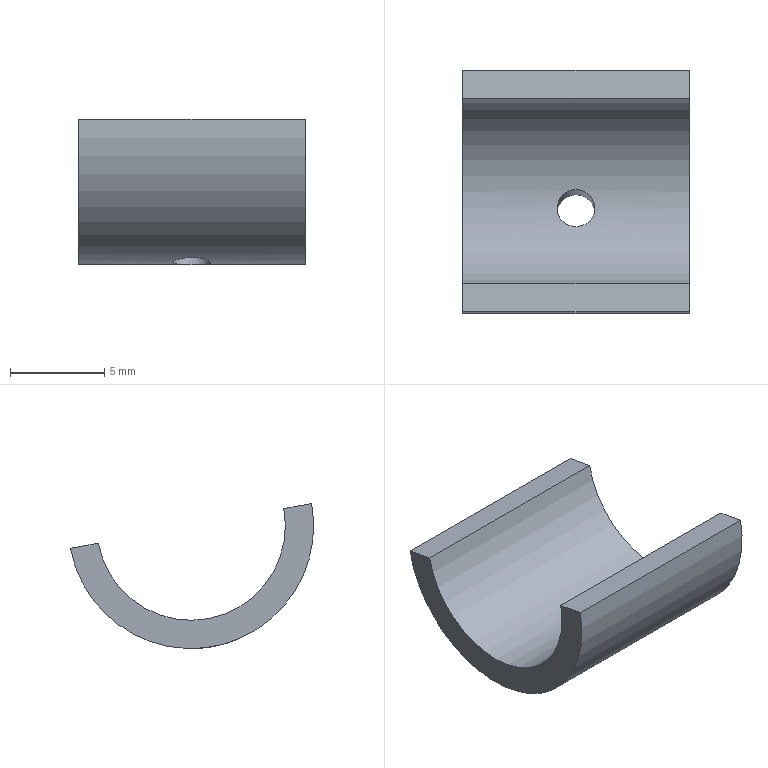Component | NX | 17C__27 | 1 solid | 7 faces | box 12 x 12.89 x 7.69 mm | volume 320 mm3 | plane 4 | cylinder 3 | commonest cylinder face diameters 10 x1 13 x1 2 x1
STEP:
#1=CARTESIAN_POINT('',(0.,0.,0.));
#2=DIRECTION('',(0.,0.,1.));
#3=DIRECTION('',(1.,0.,0.));
#4=AXIS2_PLACEMENT_3D('',#1,#2,#3);
#5=CARTESIAN_POINT('',(122.022,103.543,62.298));
#6=VERTEX_POINT('',#5);
#7=CARTESIAN_POINT('',(110.022,103.543,62.298));
#8=VERTEX_POINT('',#7);
#9=CARTESIAN_POINT('',(122.022,103.543,62.298));
#10=DIRECTION('',(-1.,0.,0.));
#11=VECTOR('',#10,1.);
#12=LINE('',#9,#11);
#13=CARTESIAN_POINT('',(122.022,98.628,63.213));
#14=DIRECTION('',(-1.,0.,0.));
#15=DIRECTION('',(0.,-0.183,-0.9831));
#16=AXIS2_PLACEMENT_3D('',#13,#14,#15);
#17=CYLINDRICAL_SURFACE('',#16,5.);
#18=CARTESIAN_POINT('',(-1.571,0.));
#19=DIRECTION('',(0.,1.));
#20=VECTOR('',#19,1.);
#21=LINE('',#18,#20);
#22=(GEOMETRIC_REPRESENTATION_CONTEXT(2)PARAMETRIC_REPRESENTATION_CONTEXT()REPRESENTATION_CONTEXT('',''));
#23=DEFINITIONAL_REPRESENTATION('',(#21),#22);
#24=PCURVE('',#17,#23);
#25=CARTESIAN_POINT('',(122.022,105.018,62.023));
#26=DIRECTION('',(0.,-0.183,-0.9831));
#27=DIRECTION('',(0.,-0.9831,0.183));
#28=AXIS2_PLACEMENT_3D('',#25,#26,#27);
#29=PLANE('',#28);
#30=CARTESIAN_POINT('',(1.5,0.));
#31=DIRECTION('',(0.,1.));
#32=VECTOR('',#31,1.);
#33=LINE('',#30,#32);
#34=(GEOMETRIC_REPRESENTATION_CONTEXT(2)PARAMETRIC_REPRESENTATION_CONTEXT()REPRESENTATION_CONTEXT('',''));
#35=DEFINITIONAL_REPRESENTATION('',(#33),#34);
#36=PCURVE('',#29,#35);
#37=SURFACE_CURVE('',#12,(#24,#36),.PCURVE_S1.);
#38=EDGE_CURVE('',#6,#8,#37,.T.);
#39=ORIENTED_EDGE('',*,*,#38,.F.);
#40=CARTESIAN_POINT('',(122.022,93.712,64.128));
#41=VERTEX_POINT('',#40);
#42=CARTESIAN_POINT('',(122.022,98.628,63.213));
#43=DIRECTION('',(-1.,0.,0.));
#44=DIRECTION('',(0.,-0.9831,0.183));
#45=AXIS2_PLACEMENT_3D('',#42,#43,#44);
#46=CIRCLE('',#45,5.);
#47=CARTESIAN_POINT('',(-4.712,0.));
#48=DIRECTION('',(1.,0.));
#49=VECTOR('',#48,1.);
#50=LINE('',#47,#49);
#51=(GEOMETRIC_REPRESENTATION_CONTEXT(2)PARAMETRIC_REPRESENTATION_CONTEXT()REPRESENTATION_CONTEXT('',''));
#52=DEFINITIONAL_REPRESENTATION('',(#50),#51);
#53=PCURVE('',#17,#52);
#54=CARTESIAN_POINT('',(122.022,98.628,63.213));
#55=DIRECTION('',(-1.,0.,0.));
#56=DIRECTION('',(0.,-0.183,-0.9831));
#57=AXIS2_PLACEMENT_3D('',#54,#55,#56);
#58=PLANE('',#57);
#59=CARTESIAN_POINT('',(0.,0.));
#60=DIRECTION('',(0.,1.));
#61=AXIS2_PLACEMENT_2D('',#59,#60);
#62=CIRCLE('',#61,5.);
#63=(GEOMETRIC_REPRESENTATION_CONTEXT(2)PARAMETRIC_REPRESENTATION_CONTEXT()REPRESENTATION_CONTEXT('',''));
#64=DEFINITIONAL_REPRESENTATION('',(#62),#63);
#65=PCURVE('',#58,#64);
#66=SURFACE_CURVE('',#46,(#53,#65),.PCURVE_S1.);
#67=EDGE_CURVE('',#6,#41,#66,.T.);
#68=ORIENTED_EDGE('',*,*,#67,.T.);
#69=CARTESIAN_POINT('',(110.022,93.712,64.128));
#70=VERTEX_POINT('',#69);
#71=CARTESIAN_POINT('',(122.022,93.712,64.128));
#72=DIRECTION('',(-1.,0.,0.));
#73=VECTOR('',#72,1.);
#74=LINE('',#71,#73);
#75=CARTESIAN_POINT('',(1.571,0.));
#76=DIRECTION('',(0.,1.));
#77=VECTOR('',#76,1.);
#78=LINE('',#75,#77);
#79=(GEOMETRIC_REPRESENTATION_CONTEXT(2)PARAMETRIC_REPRESENTATION_CONTEXT()REPRESENTATION_CONTEXT('',''));
#80=DEFINITIONAL_REPRESENTATION('',(#78),#79);
#81=PCURVE('',#17,#80);
#82=CARTESIAN_POINT('',(122.022,93.712,64.128));
#83=DIRECTION('',(0.,-0.183,-0.9831));
#84=DIRECTION('',(0.,-0.9831,0.183));
#85=AXIS2_PLACEMENT_3D('',#82,#83,#84);
#86=PLANE('',#85);
#87=CARTESIAN_POINT('',(0.,0.));
#88=DIRECTION('',(0.,1.));
#89=VECTOR('',#88,1.);
#90=LINE('',#87,#89);
#91=(GEOMETRIC_REPRESENTATION_CONTEXT(2)PARAMETRIC_REPRESENTATION_CONTEXT()REPRESENTATION_CONTEXT('',''));
#92=DEFINITIONAL_REPRESENTATION('',(#90),#91);
#93=PCURVE('',#86,#92);
#94=SURFACE_CURVE('',#74,(#81,#93),.PCURVE_S1.);
#95=EDGE_CURVE('',#41,#70,#94,.T.);
#96=ORIENTED_EDGE('',*,*,#95,.T.);
#97=CARTESIAN_POINT('',(110.022,98.628,63.213));
#98=DIRECTION('',(-1.,0.,0.));
#99=DIRECTION('',(0.,-0.9831,0.183));
#100=AXIS2_PLACEMENT_3D('',#97,#98,#99);
#101=CIRCLE('',#100,5.);
#102=CARTESIAN_POINT('',(-4.712,12.));
#103=DIRECTION('',(1.,0.));
#104=VECTOR('',#103,1.);
#105=LINE('',#102,#104);
#106=(GEOMETRIC_REPRESENTATION_CONTEXT(2)PARAMETRIC_REPRESENTATION_CONTEXT()REPRESENTATION_CONTEXT('',''));
#107=DEFINITIONAL_REPRESENTATION('',(#105),#106);
#108=PCURVE('',#17,#107);
#109=CARTESIAN_POINT('',(110.022,98.628,63.213));
#110=DIRECTION('',(-1.,0.,0.));
#111=DIRECTION('',(0.,-0.183,-0.9831));
#112=AXIS2_PLACEMENT_3D('',#109,#110,#111);
#113=PLANE('',#112);
#114=CARTESIAN_POINT('',(0.,0.));
#115=DIRECTION('',(0.,1.));
#116=AXIS2_PLACEMENT_2D('',#114,#115);
#117=CIRCLE('',#116,5.);
#118=(GEOMETRIC_REPRESENTATION_CONTEXT(2)PARAMETRIC_REPRESENTATION_CONTEXT()REPRESENTATION_CONTEXT('',''));
#119=DEFINITIONAL_REPRESENTATION('',(#117),#118);
#120=PCURVE('',#113,#119);
#121=SURFACE_CURVE('',#101,(#108,#120),.PCURVE_S1.);
#122=EDGE_CURVE('',#8,#70,#121,.T.);
#123=ORIENTED_EDGE('',*,*,#122,.F.);
#124=EDGE_LOOP('',(#39,#68,#96,#123));
#125=FACE_BOUND('',#124,.F.);
#126=CARTESIAN_POINT('',(116.022,98.714,58.213));
#127=VERTEX_POINT('',#126);
#128=CARTESIAN_POINT('',(116.022,98.714,58.213));
#129=CARTESIAN_POINT('',(115.911,98.714,58.213));
#130=CARTESIAN_POINT('',(115.799,98.695,58.213));
#131=CARTESIAN_POINT('',(115.695,98.658,58.213));
#132=CARTESIAN_POINT('',(115.591,98.621,58.212));
#133=CARTESIAN_POINT('',(115.491,98.566,58.212));
#134=CARTESIAN_POINT('',(115.405,98.497,58.214));
#135=CARTESIAN_POINT('',(115.317,98.428,58.216));
#136=CARTESIAN_POINT('',(115.24,98.342,58.22));
#137=CARTESIAN_POINT('',(115.18,98.248,58.227));
#138=CARTESIAN_POINT('',(115.119,98.153,58.234));
#139=CARTESIAN_POINT('',(115.074,98.046,58.245));
#140=CARTESIAN_POINT('',(115.048,97.937,58.26));
#141=CARTESIAN_POINT('',(115.023,97.83,58.275));
#142=CARTESIAN_POINT('',(115.016,97.717,58.295));
#143=CARTESIAN_POINT('',(115.028,97.608,58.318));
#144=CARTESIAN_POINT('',(115.039,97.501,58.34));
#145=CARTESIAN_POINT('',(115.07,97.396,58.366));
#146=CARTESIAN_POINT('',(115.116,97.3,58.392));
#147=CARTESIAN_POINT('',(115.163,97.203,58.419));
#148=CARTESIAN_POINT('',(115.227,97.113,58.447));
#149=CARTESIAN_POINT('',(115.304,97.038,58.472));
#150=CARTESIAN_POINT('',(115.382,96.961,58.498));
#151=CARTESIAN_POINT('',(115.474,96.896,58.522));
#152=CARTESIAN_POINT('',(115.575,96.848,58.54));
#153=CARTESIAN_POINT('',(115.675,96.8,58.558));
#154=CARTESIAN_POINT('',(115.786,96.769,58.571));
#155=CARTESIAN_POINT('',(115.898,96.755,58.576));
#156=CARTESIAN_POINT('',(116.008,96.742,58.582));
#157=CARTESIAN_POINT('',(116.122,96.747,58.58));
#158=CARTESIAN_POINT('',(116.23,96.769,58.571));
#159=CARTESIAN_POINT('',(116.337,96.79,58.562));
#160=CARTESIAN_POINT('',(116.442,96.829,58.547));
#161=CARTESIAN_POINT('',(116.536,96.883,58.527));
#162=CARTESIAN_POINT('',(116.631,96.937,58.507));
#163=CARTESIAN_POINT('',(116.717,97.007,58.482));
#164=CARTESIAN_POINT('',(116.788,97.089,58.455));
#165=CARTESIAN_POINT('',(116.861,97.171,58.429));
#166=CARTESIAN_POINT('',(116.919,97.267,58.4));
#167=CARTESIAN_POINT('',(116.959,97.37,58.373));
#168=CARTESIAN_POINT('',(116.998,97.472,58.347));
#169=CARTESIAN_POINT('',(117.02,97.582,58.322));
#170=CARTESIAN_POINT('',(117.022,97.692,58.301));
#171=CARTESIAN_POINT('',(117.024,97.801,58.28));
#172=CARTESIAN_POINT('',(117.008,97.912,58.263));
#173=CARTESIAN_POINT('',(116.974,98.016,58.25));
#174=CARTESIAN_POINT('',(116.94,98.12,58.237));
#175=CARTESIAN_POINT('',(116.888,98.22,58.228));
#176=CARTESIAN_POINT('',(116.823,98.308,58.223));
#177=CARTESIAN_POINT('',(116.756,98.398,58.217));
#178=CARTESIAN_POINT('',(116.673,98.478,58.214));
#179=CARTESIAN_POINT('',(116.581,98.541,58.213));
#180=CARTESIAN_POINT('',(116.488,98.604,58.212));
#181=CARTESIAN_POINT('',(116.382,98.653,58.213));
#182=CARTESIAN_POINT('',(116.273,98.682,58.213));
#183=CARTESIAN_POINT('',(116.191,98.703,58.213));
#184=CARTESIAN_POINT('',(116.106,98.714,58.213));
#185=CARTESIAN_POINT('',(116.022,98.714,58.213));
#186=B_SPLINE_CURVE_WITH_KNOTS('',3,(#128,#129,#130,#131,#132,#133,#134,#135,#136,#137,#138,#139,#140,#141,#142,#143,#144,#145,#146,#147,#148,#149,#150,#151,#152,#153,#154,#155,#156,#157,#158,#159,#160,#161,#162,#163,#164,#165,#166,#167,#168,#169,#170,#171,#172,#173,#174,#175,#176,#177,#178,#179,#180,#181,#182,#183,#184,#185),.UNSPECIFIED.,.T.,.F.,(1,3,3,3,3,3,3,3,3,3,3,3,3,3,3,3,3,3,3,3,3,1),(-0.04007,0.,0.05297,0.1059,0.1595,0.2136,0.267,0.3195,0.3725,0.4263,0.4803,0.5334,0.5859,0.6391,0.6931,0.7469,0.7997,0.8523,0.9058,0.9599,1.,1.053),.UNSPECIFIED.);
#187=CARTESIAN_POINT('',(-0.2014,6.));
#188=CARTESIAN_POINT('',(-0.2014,6.024));
#189=CARTESIAN_POINT('',(-0.201,6.071));
#190=CARTESIAN_POINT('',(-0.1994,6.143));
#191=CARTESIAN_POINT('',(-0.1968,6.213));
#192=CARTESIAN_POINT('',(-0.1932,6.283));
#193=CARTESIAN_POINT('',(-0.1886,6.35));
#194=CARTESIAN_POINT('',(-0.1831,6.416));
#195=CARTESIAN_POINT('',(-0.1765,6.48));
#196=CARTESIAN_POINT('',(-0.1691,6.542));
#197=CARTESIAN_POINT('',(-0.1609,6.6));
#198=CARTESIAN_POINT('',(-0.1519,6.655));
#199=CARTESIAN_POINT('',(-0.142,6.707));
#200=CARTESIAN_POINT('',(-0.1315,6.756));
#201=CARTESIAN_POINT('',(-0.1203,6.801));
#202=CARTESIAN_POINT('',(-0.1085,6.842));
#203=CARTESIAN_POINT('',(-0.09624,6.878));
#204=CARTESIAN_POINT('',(-0.0834,6.91));
#205=CARTESIAN_POINT('',(-0.07014,6.937));
#206=CARTESIAN_POINT('',(-0.05653,6.96));
#207=CARTESIAN_POINT('',(-0.04273,6.978));
#208=CARTESIAN_POINT('',(-0.02865,6.99));
#209=CARTESIAN_POINT('',(-0.01438,6.998));
#210=CARTESIAN_POINT('',(-0.00003491,7.001));
#211=CARTESIAN_POINT('',(0.01428,6.998));
#212=CARTESIAN_POINT('',(0.02845,6.991));
#213=CARTESIAN_POINT('',(0.04255,6.978));
#214=CARTESIAN_POINT('',(0.05647,6.96));
#215=CARTESIAN_POINT('',(0.07009,6.938));
#216=CARTESIAN_POINT('',(0.08331,6.91));
#217=CARTESIAN_POINT('',(0.09608,6.878));
#218=CARTESIAN_POINT('',(0.1084,6.842));
#219=CARTESIAN_POINT('',(0.1203,6.801));
#220=CARTESIAN_POINT('',(0.1315,6.756));
#221=CARTESIAN_POINT('',(0.142,6.708));
#222=CARTESIAN_POINT('',(0.1518,6.656));
#223=CARTESIAN_POINT('',(0.1608,6.6));
#224=CARTESIAN_POINT('',(0.1691,6.542));
#225=CARTESIAN_POINT('',(0.1765,6.48));
#226=CARTESIAN_POINT('',(0.183,6.417));
#227=CARTESIAN_POINT('',(0.1886,6.351));
#228=CARTESIAN_POINT('',(0.1932,6.283));
#229=CARTESIAN_POINT('',(0.1968,6.214));
#230=CARTESIAN_POINT('',(0.1994,6.143));
#231=CARTESIAN_POINT('',(0.201,6.072));
#232=CARTESIAN_POINT('',(0.2015,6.001));
#233=CARTESIAN_POINT('',(0.201,5.929));
#234=CARTESIAN_POINT('',(0.1994,5.858));
#235=CARTESIAN_POINT('',(0.1969,5.787));
#236=CARTESIAN_POINT('',(0.1933,5.718));
#237=CARTESIAN_POINT('',(0.1886,5.65));
#238=CARTESIAN_POINT('',(0.1831,5.584));
#239=CARTESIAN_POINT('',(0.1766,5.52));
#240=CARTESIAN_POINT('',(0.1692,5.459));
#241=CARTESIAN_POINT('',(0.161,5.401));
#242=CARTESIAN_POINT('',(0.1519,5.345));
#243=CARTESIAN_POINT('',(0.1421,5.293));
#244=CARTESIAN_POINT('',(0.1316,5.244));
#245=CARTESIAN_POINT('',(0.1204,5.2));
#246=CARTESIAN_POINT('',(0.1086,5.159));
#247=CARTESIAN_POINT('',(0.09628,5.122));
#248=CARTESIAN_POINT('',(0.08345,5.09));
#249=CARTESIAN_POINT('',(0.07026,5.063));
#250=CARTESIAN_POINT('',(0.05672,5.04));
#251=CARTESIAN_POINT('',(0.04282,5.022));
#252=CARTESIAN_POINT('',(0.02869,5.01));
#253=CARTESIAN_POINT('',(0.01444,5.002));
#254=CARTESIAN_POINT('',(0.0001984,4.999));
#255=CARTESIAN_POINT('',(-0.01411,5.002));
#256=CARTESIAN_POINT('',(-0.02838,5.009));
#257=CARTESIAN_POINT('',(-0.04251,5.022));
#258=CARTESIAN_POINT('',(-0.0564,5.04));
#259=CARTESIAN_POINT('',(-0.06992,5.062));
#260=CARTESIAN_POINT('',(-0.08318,5.09));
#261=CARTESIAN_POINT('',(-0.09603,5.122));
#262=CARTESIAN_POINT('',(-0.1084,5.158));
#263=CARTESIAN_POINT('',(-0.1202,5.198));
#264=CARTESIAN_POINT('',(-0.1313,5.243));
#265=CARTESIAN_POINT('',(-0.1419,5.292));
#266=CARTESIAN_POINT('',(-0.1517,5.344));
#267=CARTESIAN_POINT('',(-0.1608,5.399));
#268=CARTESIAN_POINT('',(-0.169,5.458));
#269=CARTESIAN_POINT('',(-0.1764,5.519));
#270=CARTESIAN_POINT('',(-0.1829,5.583));
#271=CARTESIAN_POINT('',(-0.1885,5.649));
#272=CARTESIAN_POINT('',(-0.1932,5.717));
#273=CARTESIAN_POINT('',(-0.1968,5.786));
#274=CARTESIAN_POINT('',(-0.1994,5.857));
#275=CARTESIAN_POINT('',(-0.201,5.928));
#276=CARTESIAN_POINT('',(-0.2014,5.976));
#277=CARTESIAN_POINT('',(-0.2014,6.));
#278=B_SPLINE_CURVE_WITH_KNOTS('',3,(#187,#188,#189,#190,#191,#192,#193,#194,#195,#196,#197,#198,#199,#200,#201,#202,#203,#204,#205,#206,#207,#208,#209,#210,#211,#212,#213,#214,#215,#216,#217,#218,#219,#220,#221,#222,#223,#224,#225,#226,#227,#228,#229,#230,#231,#232,#233,#234,#235,#236,#237,#238,#239,#240,#241,#242,#243,#244,#245,#246,#247,#248,#249,#250,#251,#252,#253,#254,#255,#256,#257,#258,#259,#260,#261,#262,#263,#264,#265,#266,#267,#268,#269,#270,#271,#272,#273,#274,#275,#276,#277),.UNSPECIFIED.,.T.,.F.,(4,1,1,1,1,1,1,1,1,1,1,1,1,1,1,1,1,1,1,1,1,1,1,1,1,1,1,1,1,1,1,1,1,1,1,1,1,1,1,1,1,1,1,1,1,1,1,1,1,1,1,1,1,1,1,1,1,1,1,1,1,1,1,1,1,1,1,1,1,1,1,1,1,1,1,1,1,1,1,1,1,1,1,1,1,1,1,1,4),(0.,0.01136,0.02273,0.03409,0.04545,0.05682,0.06818,0.07955,0.09091,0.1023,0.1136,0.125,0.1364,0.1477,0.1591,0.1705,0.1818,0.1932,0.2045,0.2159,0.2273,0.2386,0.25,0.2614,0.2727,0.2841,0.2955,0.3068,0.3182,0.3295,0.3409,0.3523,0.3636,0.375,0.3864,0.3977,0.4091,0.4205,0.4318,0.4432,0.4545,0.4659,0.4773,0.4886,0.5,0.5114,0.5227,0.5341,0.5455,0.5568,0.5682,0.5795,0.5909,0.6023,0.6136,0.625,0.6364,0.6477,0.6591,0.6705,0.6818,0.6932,0.7045,0.7159,0.7273,0.7386,0.75,0.7614,0.7727,0.7841,0.7955,0.8068,0.8182,0.8295,0.8409,0.8523,0.8636,0.875,0.8864,0.8977,0.9091,0.9205,0.9318,0.9432,0.9545,0.9659,0.9773,0.9886,1.),.QUASI_UNIFORM_KNOTS.);
#279=(GEOMETRIC_REPRESENTATION_CONTEXT(2)PARAMETRIC_REPRESENTATION_CONTEXT()REPRESENTATION_CONTEXT('',''));
#280=DEFINITIONAL_REPRESENTATION('',(#278),#279);
#281=PCURVE('',#17,#280);
#282=CARTESIAN_POINT('',(116.022,96.432,51.415));
#283=DIRECTION('',(0.,0.183,0.9831));
#284=DIRECTION('',(0.,0.9831,-0.183));
#285=AXIS2_PLACEMENT_3D('',#282,#283,#284);
#286=CYLINDRICAL_SURFACE('',#285,1.);
#287=CARTESIAN_POINT('',(0.,7.101));
#288=CARTESIAN_POINT('',(0.02374,7.101));
#289=CARTESIAN_POINT('',(0.07137,7.101));
#290=CARTESIAN_POINT('',(0.1431,7.099));
#291=CARTESIAN_POINT('',(0.2148,7.097));
#292=CARTESIAN_POINT('',(0.2863,7.093));
#293=CARTESIAN_POINT('',(0.3574,7.089));
#294=CARTESIAN_POINT('',(0.4288,7.084));
#295=CARTESIAN_POINT('',(0.5003,7.078));
#296=CARTESIAN_POINT('',(0.5718,7.071));
#297=CARTESIAN_POINT('',(0.643,7.065));
#298=CARTESIAN_POINT('',(0.7139,7.057));
#299=CARTESIAN_POINT('',(0.7852,7.05));
#300=CARTESIAN_POINT('',(0.8566,7.043));
#301=CARTESIAN_POINT('',(0.928,7.036));
#302=CARTESIAN_POINT('',(0.999,7.029));
#303=CARTESIAN_POINT('',(1.07,7.023));
#304=CARTESIAN_POINT('',(1.142,7.017));
#305=CARTESIAN_POINT('',(1.213,7.012));
#306=CARTESIAN_POINT('',(1.285,7.008));
#307=CARTESIAN_POINT('',(1.356,7.004));
#308=CARTESIAN_POINT('',(1.427,7.002));
#309=CARTESIAN_POINT('',(1.499,7.));
#310=CARTESIAN_POINT('',(1.571,7.));
#311=CARTESIAN_POINT('',(1.642,7.));
#312=CARTESIAN_POINT('',(1.713,7.002));
#313=CARTESIAN_POINT('',(1.785,7.004));
#314=CARTESIAN_POINT('',(1.857,7.008));
#315=CARTESIAN_POINT('',(1.928,7.012));
#316=CARTESIAN_POINT('',(2.,7.017));
#317=CARTESIAN_POINT('',(2.071,7.023));
#318=CARTESIAN_POINT('',(2.142,7.029));
#319=CARTESIAN_POINT('',(2.214,7.036));
#320=CARTESIAN_POINT('',(2.285,7.043));
#321=CARTESIAN_POINT('',(2.356,7.05));
#322=CARTESIAN_POINT('',(2.427,7.057));
#323=CARTESIAN_POINT('',(2.498,7.064));
#324=CARTESIAN_POINT('',(2.57,7.071));
#325=CARTESIAN_POINT('',(2.641,7.078));
#326=CARTESIAN_POINT('',(2.712,7.083));
#327=CARTESIAN_POINT('',(2.783,7.089));
#328=CARTESIAN_POINT('',(2.855,7.093));
#329=CARTESIAN_POINT('',(2.927,7.097));
#330=CARTESIAN_POINT('',(2.998,7.099));
#331=CARTESIAN_POINT('',(3.069,7.101));
#332=CARTESIAN_POINT('',(3.141,7.101));
#333=CARTESIAN_POINT('',(3.213,7.101));
#334=CARTESIAN_POINT('',(3.284,7.099));
#335=CARTESIAN_POINT('',(3.356,7.097));
#336=CARTESIAN_POINT('',(3.427,7.093));
#337=CARTESIAN_POINT('',(3.499,7.089));
#338=CARTESIAN_POINT('',(3.57,7.084));
#339=CARTESIAN_POINT('',(3.642,7.078));
#340=CARTESIAN_POINT('',(3.712,7.071));
#341=CARTESIAN_POINT('',(3.784,7.065));
#342=CARTESIAN_POINT('',(3.855,7.058));
#343=CARTESIAN_POINT('',(3.927,7.05));
#344=CARTESIAN_POINT('',(3.998,7.043));
#345=CARTESIAN_POINT('',(4.069,7.036));
#346=CARTESIAN_POINT('',(4.14,7.029));
#347=CARTESIAN_POINT('',(4.211,7.023));
#348=CARTESIAN_POINT('',(4.283,7.017));
#349=CARTESIAN_POINT('',(4.354,7.012));
#350=CARTESIAN_POINT('',(4.425,7.008));
#351=CARTESIAN_POINT('',(4.497,7.004));
#352=CARTESIAN_POINT('',(4.569,7.002));
#353=CARTESIAN_POINT('',(4.64,7.));
#354=CARTESIAN_POINT('',(4.711,7.));
#355=CARTESIAN_POINT('',(4.783,7.));
#356=CARTESIAN_POINT('',(4.855,7.002));
#357=CARTESIAN_POINT('',(4.926,7.004));
#358=CARTESIAN_POINT('',(4.998,7.008));
#359=CARTESIAN_POINT('',(5.069,7.012));
#360=CARTESIAN_POINT('',(5.14,7.017));
#361=CARTESIAN_POINT('',(5.212,7.023));
#362=CARTESIAN_POINT('',(5.283,7.029));
#363=CARTESIAN_POINT('',(5.355,7.036));
#364=CARTESIAN_POINT('',(5.426,7.043));
#365=CARTESIAN_POINT('',(5.497,7.05));
#366=CARTESIAN_POINT('',(5.568,7.057));
#367=CARTESIAN_POINT('',(5.64,7.064));
#368=CARTESIAN_POINT('',(5.711,7.071));
#369=CARTESIAN_POINT('',(5.782,7.078));
#370=CARTESIAN_POINT('',(5.853,7.083));
#371=CARTESIAN_POINT('',(5.925,7.089));
#372=CARTESIAN_POINT('',(5.996,7.093));
#373=CARTESIAN_POINT('',(6.067,7.097));
#374=CARTESIAN_POINT('',(6.139,7.099));
#375=CARTESIAN_POINT('',(6.211,7.101));
#376=CARTESIAN_POINT('',(6.259,7.101));
#377=CARTESIAN_POINT('',(6.283,7.101));
#378=B_SPLINE_CURVE_WITH_KNOTS('',3,(#287,#288,#289,#290,#291,#292,#293,#294,#295,#296,#297,#298,#299,#300,#301,#302,#303,#304,#305,#306,#307,#308,#309,#310,#311,#312,#313,#314,#315,#316,#317,#318,#319,#320,#321,#322,#323,#324,#325,#326,#327,#328,#329,#330,#331,#332,#333,#334,#335,#336,#337,#338,#339,#340,#341,#342,#343,#344,#345,#346,#347,#348,#349,#350,#351,#352,#353,#354,#355,#356,#357,#358,#359,#360,#361,#362,#363,#364,#365,#366,#367,#368,#369,#370,#371,#372,#373,#374,#375,#376,#377),.UNSPECIFIED.,.F.,.F.,(4,1,1,1,1,1,1,1,1,1,1,1,1,1,1,1,1,1,1,1,1,1,1,1,1,1,1,1,1,1,1,1,1,1,1,1,1,1,1,1,1,1,1,1,1,1,1,1,1,1,1,1,1,1,1,1,1,1,1,1,1,1,1,1,1,1,1,1,1,1,1,1,1,1,1,1,1,1,1,1,1,1,1,1,1,1,1,1,4),(0.,0.01136,0.02273,0.03409,0.04545,0.05682,0.06818,0.07955,0.09091,0.1023,0.1136,0.125,0.1364,0.1477,0.1591,0.1705,0.1818,0.1932,0.2045,0.2159,0.2273,0.2386,0.25,0.2614,0.2727,0.2841,0.2955,0.3068,0.3182,0.3295,0.3409,0.3523,0.3636,0.375,0.3864,0.3977,0.4091,0.4205,0.4318,0.4432,0.4545,0.4659,0.4773,0.4886,0.5,0.5114,0.5227,0.5341,0.5455,0.5568,0.5682,0.5795,0.5909,0.6023,0.6136,0.625,0.6364,0.6477,0.6591,0.6705,0.6818,0.6932,0.7045,0.7159,0.7273,0.7386,0.75,0.7614,0.7727,0.7841,0.7955,0.8068,0.8182,0.8295,0.8409,0.8523,0.8636,0.875,0.8864,0.8977,0.9091,0.9205,0.9318,0.9432,0.9545,0.9659,0.9773,0.9886,1.),.QUASI_UNIFORM_KNOTS.);
#379=(GEOMETRIC_REPRESENTATION_CONTEXT(2)PARAMETRIC_REPRESENTATION_CONTEXT()REPRESENTATION_CONTEXT('',''));
#380=DEFINITIONAL_REPRESENTATION('',(#378),#379);
#381=PCURVE('',#286,#380);
#382=SURFACE_CURVE('',#186,(#281,#381),.PCURVE_S1.);
#383=EDGE_CURVE('',#127,#127,#382,.T.);
#384=ORIENTED_EDGE('',*,*,#383,.T.);
#385=EDGE_LOOP('',(#384));
#386=FACE_BOUND('',#385,.F.);
#387=ADVANCED_FACE('',(#125,#386),#17,.F.);
#388=CARTESIAN_POINT('',(110.022,92.237,64.402));
#389=VERTEX_POINT('',#388);
#390=CARTESIAN_POINT('',(110.022,105.018,62.023));
#391=VERTEX_POINT('',#390);
#392=CARTESIAN_POINT('',(110.022,98.628,63.213));
#393=DIRECTION('',(1.,0.,0.));
#394=DIRECTION('',(0.,-0.9831,0.183));
#395=AXIS2_PLACEMENT_3D('',#392,#393,#394);
#396=CIRCLE('',#395,6.5);
#397=CARTESIAN_POINT('',(122.022,98.628,63.213));
#398=DIRECTION('',(-1.,0.,0.));
#399=DIRECTION('',(0.,-0.183,-0.9831));
#400=AXIS2_PLACEMENT_3D('',#397,#398,#399);
#401=CYLINDRICAL_SURFACE('',#400,6.5);
#402=CARTESIAN_POINT('',(1.571,12.));
#403=DIRECTION('',(-1.,0.));
#404=VECTOR('',#403,1.);
#405=LINE('',#402,#404);
#406=(GEOMETRIC_REPRESENTATION_CONTEXT(2)PARAMETRIC_REPRESENTATION_CONTEXT()REPRESENTATION_CONTEXT('',''));
#407=DEFINITIONAL_REPRESENTATION('',(#405),#406);
#408=PCURVE('',#401,#407);
#409=CARTESIAN_POINT('',(0.,6.5));
#410=CARTESIAN_POINT('',(11.258,6.5));
#411=CARTESIAN_POINT('',(5.629,-3.25));
#412=CARTESIAN_POINT('',(0.,-13.));
#413=CARTESIAN_POINT('',(-5.629,-3.25));
#414=CARTESIAN_POINT('',(-11.258,6.5));
#415=CARTESIAN_POINT('',(0.,6.5));
#416=(BOUNDED_CURVE()B_SPLINE_CURVE(2,(#409,#410,#411,#412,#413,#414,#415),.UNSPECIFIED.,.T.,.F.)B_SPLINE_CURVE_WITH_KNOTS((1,2,2,2,2,1),(-2.094,0.,2.094,4.189,6.283,8.378),.UNSPECIFIED.)CURVE()GEOMETRIC_REPRESENTATION_ITEM()RATIONAL_B_SPLINE_CURVE((1.,0.5,1.,0.5,1.,0.5,1.))REPRESENTATION_ITEM(''));
#417=(GEOMETRIC_REPRESENTATION_CONTEXT(2)PARAMETRIC_REPRESENTATION_CONTEXT()REPRESENTATION_CONTEXT('',''));
#418=DEFINITIONAL_REPRESENTATION('',(#416),#417);
#419=PCURVE('',#113,#418);
#420=SURFACE_CURVE('',#396,(#408,#419),.PCURVE_S1.);
#421=EDGE_CURVE('',#389,#391,#420,.T.);
#422=ORIENTED_EDGE('',*,*,#421,.T.);
#423=CARTESIAN_POINT('',(122.022,105.018,62.023));
#424=VERTEX_POINT('',#423);
#425=CARTESIAN_POINT('',(122.022,105.018,62.023));
#426=DIRECTION('',(-1.,0.,0.));
#427=VECTOR('',#426,1.);
#428=LINE('',#425,#427);
#429=CARTESIAN_POINT('',(-1.571,0.));
#430=DIRECTION('',(0.,1.));
#431=VECTOR('',#430,1.);
#432=LINE('',#429,#431);
#433=(GEOMETRIC_REPRESENTATION_CONTEXT(2)PARAMETRIC_REPRESENTATION_CONTEXT()REPRESENTATION_CONTEXT('',''));
#434=DEFINITIONAL_REPRESENTATION('',(#432),#433);
#435=PCURVE('',#401,#434);
#436=CARTESIAN_POINT('',(0.,0.));
#437=DIRECTION('',(0.,1.));
#438=VECTOR('',#437,1.);
#439=LINE('',#436,#438);
#440=(GEOMETRIC_REPRESENTATION_CONTEXT(2)PARAMETRIC_REPRESENTATION_CONTEXT()REPRESENTATION_CONTEXT('',''));
#441=DEFINITIONAL_REPRESENTATION('',(#439),#440);
#442=PCURVE('',#29,#441);
#443=SURFACE_CURVE('',#428,(#435,#442),.PCURVE_S1.);
#444=EDGE_CURVE('',#424,#391,#443,.T.);
#445=ORIENTED_EDGE('',*,*,#444,.F.);
#446=CARTESIAN_POINT('',(122.022,92.237,64.402));
#447=VERTEX_POINT('',#446);
#448=CARTESIAN_POINT('',(122.022,98.628,63.213));
#449=DIRECTION('',(1.,0.,0.));
#450=DIRECTION('',(0.,-0.9831,0.183));
#451=AXIS2_PLACEMENT_3D('',#448,#449,#450);
#452=CIRCLE('',#451,6.5);
#453=CARTESIAN_POINT('',(1.571,0.));
#454=DIRECTION('',(-1.,0.));
#455=VECTOR('',#454,1.);
#456=LINE('',#453,#455);
#457=(GEOMETRIC_REPRESENTATION_CONTEXT(2)PARAMETRIC_REPRESENTATION_CONTEXT()REPRESENTATION_CONTEXT('',''));
#458=DEFINITIONAL_REPRESENTATION('',(#456),#457);
#459=PCURVE('',#401,#458);
#460=CARTESIAN_POINT('',(0.,6.5));
#461=CARTESIAN_POINT('',(11.258,6.5));
#462=CARTESIAN_POINT('',(5.629,-3.25));
#463=CARTESIAN_POINT('',(0.,-13.));
#464=CARTESIAN_POINT('',(-5.629,-3.25));
#465=CARTESIAN_POINT('',(-11.258,6.5));
#466=CARTESIAN_POINT('',(0.,6.5));
#467=(BOUNDED_CURVE()B_SPLINE_CURVE(2,(#460,#461,#462,#463,#464,#465,#466),.UNSPECIFIED.,.T.,.F.)B_SPLINE_CURVE_WITH_KNOTS((1,2,2,2,2,1),(-2.094,0.,2.094,4.189,6.283,8.378),.UNSPECIFIED.)CURVE()GEOMETRIC_REPRESENTATION_ITEM()RATIONAL_B_SPLINE_CURVE((1.,0.5,1.,0.5,1.,0.5,1.))REPRESENTATION_ITEM(''));
#468=(GEOMETRIC_REPRESENTATION_CONTEXT(2)PARAMETRIC_REPRESENTATION_CONTEXT()REPRESENTATION_CONTEXT('',''));
#469=DEFINITIONAL_REPRESENTATION('',(#467),#468);
#470=PCURVE('',#58,#469);
#471=SURFACE_CURVE('',#452,(#459,#470),.PCURVE_S1.);
#472=EDGE_CURVE('',#447,#424,#471,.T.);
#473=ORIENTED_EDGE('',*,*,#472,.F.);
#474=CARTESIAN_POINT('',(122.022,92.237,64.402));
#475=DIRECTION('',(-1.,0.,0.));
#476=VECTOR('',#475,1.);
#477=LINE('',#474,#476);
#478=CARTESIAN_POINT('',(1.571,0.));
#479=DIRECTION('',(0.,1.));
#480=VECTOR('',#479,1.);
#481=LINE('',#478,#480);
#482=(GEOMETRIC_REPRESENTATION_CONTEXT(2)PARAMETRIC_REPRESENTATION_CONTEXT()REPRESENTATION_CONTEXT('',''));
#483=DEFINITIONAL_REPRESENTATION('',(#481),#482);
#484=PCURVE('',#401,#483);
#485=CARTESIAN_POINT('',(1.5,0.));
#486=DIRECTION('',(0.,1.));
#487=VECTOR('',#486,1.);
#488=LINE('',#485,#487);
#489=(GEOMETRIC_REPRESENTATION_CONTEXT(2)PARAMETRIC_REPRESENTATION_CONTEXT()REPRESENTATION_CONTEXT('',''));
#490=DEFINITIONAL_REPRESENTATION('',(#488),#489);
#491=PCURVE('',#86,#490);
#492=SURFACE_CURVE('',#477,(#484,#491),.PCURVE_S1.);
#493=EDGE_CURVE('',#447,#389,#492,.T.);
#494=ORIENTED_EDGE('',*,*,#493,.T.);
#495=EDGE_LOOP('',(#422,#445,#473,#494));
#496=FACE_BOUND('',#495,.T.);
#497=CARTESIAN_POINT('',(116.022,98.435,56.715));
#498=VERTEX_POINT('',#497);
#499=CARTESIAN_POINT('',(116.022,98.435,56.715));
#500=CARTESIAN_POINT('',(116.133,98.435,56.715));
#501=CARTESIAN_POINT('',(116.246,98.416,56.716));
#502=CARTESIAN_POINT('',(116.351,98.379,56.717));
#503=CARTESIAN_POINT('',(116.456,98.342,56.719));
#504=CARTESIAN_POINT('',(116.556,98.287,56.721));
#505=CARTESIAN_POINT('',(116.643,98.218,56.726));
#506=CARTESIAN_POINT('',(116.73,98.148,56.73));
#507=CARTESIAN_POINT('',(116.807,98.063,56.736));
#508=CARTESIAN_POINT('',(116.867,97.968,56.746));
#509=CARTESIAN_POINT('',(116.927,97.874,56.756));
#510=CARTESIAN_POINT('',(116.971,97.768,56.769));
#511=CARTESIAN_POINT('',(116.997,97.659,56.785));
#512=CARTESIAN_POINT('',(117.022,97.552,56.801));
#513=CARTESIAN_POINT('',(117.028,97.439,56.821));
#514=CARTESIAN_POINT('',(117.016,97.33,56.843));
#515=CARTESIAN_POINT('',(117.004,97.222,56.865));
#516=CARTESIAN_POINT('',(116.973,97.116,56.89));
#517=CARTESIAN_POINT('',(116.925,97.019,56.915));
#518=CARTESIAN_POINT('',(116.878,96.921,56.94));
#519=CARTESIAN_POINT('',(116.812,96.831,56.965));
#520=CARTESIAN_POINT('',(116.735,96.755,56.988));
#521=CARTESIAN_POINT('',(116.656,96.678,57.011));
#522=CARTESIAN_POINT('',(116.562,96.614,57.032));
#523=CARTESIAN_POINT('',(116.462,96.567,57.048));
#524=CARTESIAN_POINT('',(116.361,96.519,57.064));
#525=CARTESIAN_POINT('',(116.25,96.488,57.075));
#526=CARTESIAN_POINT('',(116.139,96.476,57.079));
#527=CARTESIAN_POINT('',(116.028,96.463,57.083));
#528=CARTESIAN_POINT('',(115.914,96.469,57.081));
#529=CARTESIAN_POINT('',(115.805,96.492,57.073));
#530=CARTESIAN_POINT('',(115.697,96.515,57.066));
#531=CARTESIAN_POINT('',(115.592,96.556,57.051));
#532=CARTESIAN_POINT('',(115.498,96.611,57.033));
#533=CARTESIAN_POINT('',(115.403,96.667,57.015));
#534=CARTESIAN_POINT('',(115.317,96.739,56.992));
#535=CARTESIAN_POINT('',(115.247,96.823,56.968));
#536=CARTESIAN_POINT('',(115.176,96.907,56.944));
#537=CARTESIAN_POINT('',(115.119,97.004,56.918));
#538=CARTESIAN_POINT('',(115.081,97.107,56.893));
#539=CARTESIAN_POINT('',(115.043,97.209,56.868));
#540=CARTESIAN_POINT('',(115.023,97.32,56.844));
#541=CARTESIAN_POINT('',(115.022,97.43,56.824));
#542=CARTESIAN_POINT('',(115.021,97.539,56.803));
#543=CARTESIAN_POINT('',(115.039,97.651,56.786));
#544=CARTESIAN_POINT('',(115.075,97.755,56.771));
#545=CARTESIAN_POINT('',(115.11,97.859,56.757));
#546=CARTESIAN_POINT('',(115.164,97.959,56.746));
#547=CARTESIAN_POINT('',(115.232,98.046,56.739));
#548=CARTESIAN_POINT('',(115.3,98.134,56.731));
#549=CARTESIAN_POINT('',(115.385,98.212,56.726));
#550=CARTESIAN_POINT('',(115.479,98.273,56.722));
#551=CARTESIAN_POINT('',(115.573,98.335,56.719));
#552=CARTESIAN_POINT('',(115.679,98.381,56.717));
#553=CARTESIAN_POINT('',(115.788,98.407,56.716));
#554=CARTESIAN_POINT('',(115.865,98.426,56.716));
#555=CARTESIAN_POINT('',(115.944,98.435,56.715));
#556=CARTESIAN_POINT('',(116.022,98.435,56.715));
#557=B_SPLINE_CURVE_WITH_KNOTS('',3,(#499,#500,#501,#502,#503,#504,#505,#506,#507,#508,#509,#510,#511,#512,#513,#514,#515,#516,#517,#518,#519,#520,#521,#522,#523,#524,#525,#526,#527,#528,#529,#530,#531,#532,#533,#534,#535,#536,#537,#538,#539,#540,#541,#542,#543,#544,#545,#546,#547,#548,#549,#550,#551,#552,#553,#554,#555,#556),.UNSPECIFIED.,.T.,.F.,(1,3,3,3,3,3,3,3,3,3,3,3,3,3,3,3,3,3,3,3,3,1),(-0.03731,0.,0.05327,0.1065,0.1602,0.2141,0.2676,0.3206,0.3739,0.4277,0.4815,0.5348,0.5878,0.6413,0.6952,0.7489,0.802,0.8551,0.9088,0.9627,1.,1.053),.UNSPECIFIED.);
#558=CARTESIAN_POINT('',(-0.1545,6.));
#559=CARTESIAN_POINT('',(-0.1545,5.976));
#560=CARTESIAN_POINT('',(-0.1542,5.929));
#561=CARTESIAN_POINT('',(-0.153,5.857));
#562=CARTESIAN_POINT('',(-0.151,5.787));
#563=CARTESIAN_POINT('',(-0.1483,5.718));
#564=CARTESIAN_POINT('',(-0.1448,5.65));
#565=CARTESIAN_POINT('',(-0.1405,5.584));
#566=CARTESIAN_POINT('',(-0.1355,5.52));
#567=CARTESIAN_POINT('',(-0.1299,5.459));
#568=CARTESIAN_POINT('',(-0.1236,5.4));
#569=CARTESIAN_POINT('',(-0.1166,5.345));
#570=CARTESIAN_POINT('',(-0.1091,5.293));
#571=CARTESIAN_POINT('',(-0.101,5.244));
#572=CARTESIAN_POINT('',(-0.09242,5.199));
#573=CARTESIAN_POINT('',(-0.08339,5.158));
#574=CARTESIAN_POINT('',(-0.07396,5.122));
#575=CARTESIAN_POINT('',(-0.06409,5.09));
#576=CARTESIAN_POINT('',(-0.0539,5.063));
#577=CARTESIAN_POINT('',(-0.04344,5.04));
#578=CARTESIAN_POINT('',(-0.03283,5.022));
#579=CARTESIAN_POINT('',(-0.02202,5.009));
#580=CARTESIAN_POINT('',(-0.01105,5.002));
#581=CARTESIAN_POINT('',(-0.00002705,4.999));
#582=CARTESIAN_POINT('',(0.01098,5.002));
#583=CARTESIAN_POINT('',(0.02186,5.009));
#584=CARTESIAN_POINT('',(0.0327,5.022));
#585=CARTESIAN_POINT('',(0.04339,5.04));
#586=CARTESIAN_POINT('',(0.05386,5.062));
#587=CARTESIAN_POINT('',(0.06402,5.09));
#588=CARTESIAN_POINT('',(0.07382,5.121));
#589=CARTESIAN_POINT('',(0.08331,5.158));
#590=CARTESIAN_POINT('',(0.09238,5.199));
#591=CARTESIAN_POINT('',(0.101,5.244));
#592=CARTESIAN_POINT('',(0.109,5.292));
#593=CARTESIAN_POINT('',(0.1166,5.344));
#594=CARTESIAN_POINT('',(0.1235,5.4));
#595=CARTESIAN_POINT('',(0.1298,5.458));
#596=CARTESIAN_POINT('',(0.1355,5.52));
#597=CARTESIAN_POINT('',(0.1405,5.583));
#598=CARTESIAN_POINT('',(0.1447,5.649));
#599=CARTESIAN_POINT('',(0.1482,5.717));
#600=CARTESIAN_POINT('',(0.151,5.787));
#601=CARTESIAN_POINT('',(0.153,5.857));
#602=CARTESIAN_POINT('',(0.1542,5.928));
#603=CARTESIAN_POINT('',(0.1546,5.999));
#604=CARTESIAN_POINT('',(0.1542,6.071));
#605=CARTESIAN_POINT('',(0.153,6.142));
#606=CARTESIAN_POINT('',(0.151,6.212));
#607=CARTESIAN_POINT('',(0.1483,6.281));
#608=CARTESIAN_POINT('',(0.1448,6.349));
#609=CARTESIAN_POINT('',(0.1405,6.416));
#610=CARTESIAN_POINT('',(0.1356,6.48));
#611=CARTESIAN_POINT('',(0.1299,6.541));
#612=CARTESIAN_POINT('',(0.1236,6.599));
#613=CARTESIAN_POINT('',(0.1167,6.655));
#614=CARTESIAN_POINT('',(0.1091,6.707));
#615=CARTESIAN_POINT('',(0.1011,6.756));
#616=CARTESIAN_POINT('',(0.09254,6.801));
#617=CARTESIAN_POINT('',(0.08348,6.841));
#618=CARTESIAN_POINT('',(0.07399,6.878));
#619=CARTESIAN_POINT('',(0.06413,6.91));
#620=CARTESIAN_POINT('',(0.05399,6.937));
#621=CARTESIAN_POINT('',(0.0436,6.96));
#622=CARTESIAN_POINT('',(0.03291,6.978));
#623=CARTESIAN_POINT('',(0.02206,6.99));
#624=CARTESIAN_POINT('',(0.0111,6.998));
#625=CARTESIAN_POINT('',(0.0001469,7.001));
#626=CARTESIAN_POINT('',(-0.01083,6.998));
#627=CARTESIAN_POINT('',(-0.0218,6.991));
#628=CARTESIAN_POINT('',(-0.03266,6.978));
#629=CARTESIAN_POINT('',(-0.04334,6.96));
#630=CARTESIAN_POINT('',(-0.05373,6.938));
#631=CARTESIAN_POINT('',(-0.0639,6.911));
#632=CARTESIAN_POINT('',(-0.07377,6.879));
#633=CARTESIAN_POINT('',(-0.08327,6.842));
#634=CARTESIAN_POINT('',(-0.09233,6.802));
#635=CARTESIAN_POINT('',(-0.1009,6.757));
#636=CARTESIAN_POINT('',(-0.109,6.708));
#637=CARTESIAN_POINT('',(-0.1165,6.656));
#638=CARTESIAN_POINT('',(-0.1235,6.601));
#639=CARTESIAN_POINT('',(-0.1298,6.542));
#640=CARTESIAN_POINT('',(-0.1354,6.481));
#641=CARTESIAN_POINT('',(-0.1404,6.417));
#642=CARTESIAN_POINT('',(-0.1447,6.351));
#643=CARTESIAN_POINT('',(-0.1482,6.283));
#644=CARTESIAN_POINT('',(-0.151,6.214));
#645=CARTESIAN_POINT('',(-0.153,6.143));
#646=CARTESIAN_POINT('',(-0.1542,6.072));
#647=CARTESIAN_POINT('',(-0.1545,6.024));
#648=CARTESIAN_POINT('',(-0.1545,6.));
#649=B_SPLINE_CURVE_WITH_KNOTS('',3,(#558,#559,#560,#561,#562,#563,#564,#565,#566,#567,#568,#569,#570,#571,#572,#573,#574,#575,#576,#577,#578,#579,#580,#581,#582,#583,#584,#585,#586,#587,#588,#589,#590,#591,#592,#593,#594,#595,#596,#597,#598,#599,#600,#601,#602,#603,#604,#605,#606,#607,#608,#609,#610,#611,#612,#613,#614,#615,#616,#617,#618,#619,#620,#621,#622,#623,#624,#625,#626,#627,#628,#629,#630,#631,#632,#633,#634,#635,#636,#637,#638,#639,#640,#641,#642,#643,#644,#645,#646,#647,#648),.UNSPECIFIED.,.T.,.F.,(4,1,1,1,1,1,1,1,1,1,1,1,1,1,1,1,1,1,1,1,1,1,1,1,1,1,1,1,1,1,1,1,1,1,1,1,1,1,1,1,1,1,1,1,1,1,1,1,1,1,1,1,1,1,1,1,1,1,1,1,1,1,1,1,1,1,1,1,1,1,1,1,1,1,1,1,1,1,1,1,1,1,1,1,1,1,1,1,4),(0.,0.01136,0.02273,0.03409,0.04545,0.05682,0.06818,0.07955,0.09091,0.1023,0.1136,0.125,0.1364,0.1477,0.1591,0.1705,0.1818,0.1932,0.2045,0.2159,0.2273,0.2386,0.25,0.2614,0.2727,0.2841,0.2955,0.3068,0.3182,0.3295,0.3409,0.3523,0.3636,0.375,0.3864,0.3977,0.4091,0.4205,0.4318,0.4432,0.4545,0.4659,0.4773,0.4886,0.5,0.5114,0.5227,0.5341,0.5455,0.5568,0.5682,0.5795,0.5909,0.6023,0.6136,0.625,0.6364,0.6477,0.6591,0.6705,0.6818,0.6932,0.7045,0.7159,0.7273,0.7386,0.75,0.7614,0.7727,0.7841,0.7955,0.8068,0.8182,0.8295,0.8409,0.8523,0.8636,0.875,0.8864,0.8977,0.9091,0.9205,0.9318,0.9432,0.9545,0.9659,0.9773,0.9886,1.),.QUASI_UNIFORM_KNOTS.);
#650=(GEOMETRIC_REPRESENTATION_CONTEXT(2)PARAMETRIC_REPRESENTATION_CONTEXT()REPRESENTATION_CONTEXT('',''));
#651=DEFINITIONAL_REPRESENTATION('',(#649),#650);
#652=PCURVE('',#401,#651);
#653=CARTESIAN_POINT('',(6.283,5.577));
#654=CARTESIAN_POINT('',(6.259,5.577));
#655=CARTESIAN_POINT('',(6.212,5.577));
#656=CARTESIAN_POINT('',(6.14,5.576));
#657=CARTESIAN_POINT('',(6.069,5.574));
#658=CARTESIAN_POINT('',(5.997,5.571));
#659=CARTESIAN_POINT('',(5.926,5.568));
#660=CARTESIAN_POINT('',(5.855,5.564));
#661=CARTESIAN_POINT('',(5.783,5.56));
#662=CARTESIAN_POINT('',(5.712,5.555));
#663=CARTESIAN_POINT('',(5.64,5.55));
#664=CARTESIAN_POINT('',(5.569,5.544));
#665=CARTESIAN_POINT('',(5.498,5.539));
#666=CARTESIAN_POINT('',(5.427,5.533));
#667=CARTESIAN_POINT('',(5.355,5.528));
#668=CARTESIAN_POINT('',(5.284,5.522));
#669=CARTESIAN_POINT('',(5.213,5.518));
#670=CARTESIAN_POINT('',(5.141,5.513));
#671=CARTESIAN_POINT('',(5.07,5.509));
#672=CARTESIAN_POINT('',(4.998,5.506));
#673=CARTESIAN_POINT('',(4.927,5.503));
#674=CARTESIAN_POINT('',(4.856,5.501));
#675=CARTESIAN_POINT('',(4.784,5.5));
#676=CARTESIAN_POINT('',(4.713,5.5));
#677=CARTESIAN_POINT('',(4.641,5.5));
#678=CARTESIAN_POINT('',(4.57,5.501));
#679=CARTESIAN_POINT('',(4.498,5.503));
#680=CARTESIAN_POINT('',(4.427,5.506));
#681=CARTESIAN_POINT('',(4.355,5.509));
#682=CARTESIAN_POINT('',(4.284,5.513));
#683=CARTESIAN_POINT('',(4.213,5.518));
#684=CARTESIAN_POINT('',(4.141,5.522));
#685=CARTESIAN_POINT('',(4.07,5.528));
#686=CARTESIAN_POINT('',(3.998,5.533));
#687=CARTESIAN_POINT('',(3.927,5.539));
#688=CARTESIAN_POINT('',(3.856,5.544));
#689=CARTESIAN_POINT('',(3.785,5.549));
#690=CARTESIAN_POINT('',(3.713,5.555));
#691=CARTESIAN_POINT('',(3.642,5.56));
#692=CARTESIAN_POINT('',(3.571,5.564));
#693=CARTESIAN_POINT('',(3.5,5.568));
#694=CARTESIAN_POINT('',(3.428,5.571));
#695=CARTESIAN_POINT('',(3.356,5.574));
#696=CARTESIAN_POINT('',(3.285,5.576));
#697=CARTESIAN_POINT('',(3.214,5.577));
#698=CARTESIAN_POINT('',(3.142,5.577));
#699=CARTESIAN_POINT('',(3.071,5.577));
#700=CARTESIAN_POINT('',(2.999,5.576));
#701=CARTESIAN_POINT('',(2.928,5.574));
#702=CARTESIAN_POINT('',(2.857,5.571));
#703=CARTESIAN_POINT('',(2.785,5.568));
#704=CARTESIAN_POINT('',(2.713,5.564));
#705=CARTESIAN_POINT('',(2.642,5.56));
#706=CARTESIAN_POINT('',(2.571,5.555));
#707=CARTESIAN_POINT('',(2.5,5.55));
#708=CARTESIAN_POINT('',(2.428,5.544));
#709=CARTESIAN_POINT('',(2.357,5.539));
#710=CARTESIAN_POINT('',(2.285,5.533));
#711=CARTESIAN_POINT('',(2.215,5.528));
#712=CARTESIAN_POINT('',(2.143,5.523));
#713=CARTESIAN_POINT('',(2.072,5.518));
#714=CARTESIAN_POINT('',(2.,5.513));
#715=CARTESIAN_POINT('',(1.929,5.509));
#716=CARTESIAN_POINT('',(1.858,5.506));
#717=CARTESIAN_POINT('',(1.786,5.503));
#718=CARTESIAN_POINT('',(1.715,5.501));
#719=CARTESIAN_POINT('',(1.643,5.5));
#720=CARTESIAN_POINT('',(1.572,5.5));
#721=CARTESIAN_POINT('',(1.5,5.5));
#722=CARTESIAN_POINT('',(1.429,5.501));
#723=CARTESIAN_POINT('',(1.357,5.503));
#724=CARTESIAN_POINT('',(1.286,5.506));
#725=CARTESIAN_POINT('',(1.215,5.509));
#726=CARTESIAN_POINT('',(1.143,5.513));
#727=CARTESIAN_POINT('',(1.072,5.518));
#728=CARTESIAN_POINT('',(1.,5.522));
#729=CARTESIAN_POINT('',(0.9288,5.528));
#730=CARTESIAN_POINT('',(0.8579,5.533));
#731=CARTESIAN_POINT('',(0.7865,5.538));
#732=CARTESIAN_POINT('',(0.715,5.544));
#733=CARTESIAN_POINT('',(0.6436,5.549));
#734=CARTESIAN_POINT('',(0.5725,5.555));
#735=CARTESIAN_POINT('',(0.5014,5.559));
#736=CARTESIAN_POINT('',(0.4299,5.564));
#737=CARTESIAN_POINT('',(0.3583,5.568));
#738=CARTESIAN_POINT('',(0.2868,5.571));
#739=CARTESIAN_POINT('',(0.2157,5.574));
#740=CARTESIAN_POINT('',(0.1437,5.576));
#741=CARTESIAN_POINT('',(0.07178,5.577));
#742=CARTESIAN_POINT('',(0.02389,5.577));
#743=CARTESIAN_POINT('',(0.,5.577));
#744=B_SPLINE_CURVE_WITH_KNOTS('',3,(#653,#654,#655,#656,#657,#658,#659,#660,#661,#662,#663,#664,#665,#666,#667,#668,#669,#670,#671,#672,#673,#674,#675,#676,#677,#678,#679,#680,#681,#682,#683,#684,#685,#686,#687,#688,#689,#690,#691,#692,#693,#694,#695,#696,#697,#698,#699,#700,#701,#702,#703,#704,#705,#706,#707,#708,#709,#710,#711,#712,#713,#714,#715,#716,#717,#718,#719,#720,#721,#722,#723,#724,#725,#726,#727,#728,#729,#730,#731,#732,#733,#734,#735,#736,#737,#738,#739,#740,#741,#742,#743),.UNSPECIFIED.,.F.,.F.,(4,1,1,1,1,1,1,1,1,1,1,1,1,1,1,1,1,1,1,1,1,1,1,1,1,1,1,1,1,1,1,1,1,1,1,1,1,1,1,1,1,1,1,1,1,1,1,1,1,1,1,1,1,1,1,1,1,1,1,1,1,1,1,1,1,1,1,1,1,1,1,1,1,1,1,1,1,1,1,1,1,1,1,1,1,1,1,1,4),(0.,0.01136,0.02273,0.03409,0.04545,0.05682,0.06818,0.07955,0.09091,0.1023,0.1136,0.125,0.1364,0.1477,0.1591,0.1705,0.1818,0.1932,0.2045,0.2159,0.2273,0.2386,0.25,0.2614,0.2727,0.2841,0.2955,0.3068,0.3182,0.3295,0.3409,0.3523,0.3636,0.375,0.3864,0.3977,0.4091,0.4205,0.4318,0.4432,0.4545,0.4659,0.4773,0.4886,0.5,0.5114,0.5227,0.5341,0.5455,0.5568,0.5682,0.5795,0.5909,0.6023,0.6136,0.625,0.6364,0.6477,0.6591,0.6705,0.6818,0.6932,0.7045,0.7159,0.7273,0.7386,0.75,0.7614,0.7727,0.7841,0.7955,0.8068,0.8182,0.8295,0.8409,0.8523,0.8636,0.875,0.8864,0.8977,0.9091,0.9205,0.9318,0.9432,0.9545,0.9659,0.9773,0.9886,1.),.QUASI_UNIFORM_KNOTS.);
#745=(GEOMETRIC_REPRESENTATION_CONTEXT(2)PARAMETRIC_REPRESENTATION_CONTEXT()REPRESENTATION_CONTEXT('',''));
#746=DEFINITIONAL_REPRESENTATION('',(#744),#745);
#747=PCURVE('',#286,#746);
#748=SURFACE_CURVE('',#557,(#652,#747),.PCURVE_S1.);
#749=EDGE_CURVE('',#498,#498,#748,.T.);
#750=ORIENTED_EDGE('',*,*,#749,.F.);
#751=EDGE_LOOP('',(#750));
#752=FACE_BOUND('',#751,.T.);
#753=ADVANCED_FACE('',(#496,#752),#401,.T.);
#754=CARTESIAN_POINT('',(110.022,105.018,62.023));
#755=DIRECTION('',(0.,-0.9831,0.183));
#756=VECTOR('',#755,1.);
#757=LINE('',#754,#756);
#758=CARTESIAN_POINT('',(0.,12.));
#759=DIRECTION('',(1.,0.));
#760=VECTOR('',#759,1.);
#761=LINE('',#758,#760);
#762=(GEOMETRIC_REPRESENTATION_CONTEXT(2)PARAMETRIC_REPRESENTATION_CONTEXT()REPRESENTATION_CONTEXT('',''));
#763=DEFINITIONAL_REPRESENTATION('',(#761),#762);
#764=PCURVE('',#29,#763);
#765=CARTESIAN_POINT('',(0.,-6.5));
#766=DIRECTION('',(0.,1.));
#767=VECTOR('',#766,1.);
#768=LINE('',#765,#767);
#769=(GEOMETRIC_REPRESENTATION_CONTEXT(2)PARAMETRIC_REPRESENTATION_CONTEXT()REPRESENTATION_CONTEXT('',''));
#770=DEFINITIONAL_REPRESENTATION('',(#768),#769);
#771=PCURVE('',#113,#770);
#772=SURFACE_CURVE('',#757,(#764,#771),.PCURVE_S1.);
#773=EDGE_CURVE('',#391,#8,#772,.T.);
#774=ORIENTED_EDGE('',*,*,#773,.T.);
#775=ORIENTED_EDGE('',*,*,#38,.F.);
#776=CARTESIAN_POINT('',(122.022,105.018,62.023));
#777=DIRECTION('',(0.,-0.9831,0.183));
#778=VECTOR('',#777,1.);
#779=LINE('',#776,#778);
#780=CARTESIAN_POINT('',(0.,0.));
#781=DIRECTION('',(1.,0.));
#782=VECTOR('',#781,1.);
#783=LINE('',#780,#782);
#784=(GEOMETRIC_REPRESENTATION_CONTEXT(2)PARAMETRIC_REPRESENTATION_CONTEXT()REPRESENTATION_CONTEXT('',''));
#785=DEFINITIONAL_REPRESENTATION('',(#783),#784);
#786=PCURVE('',#29,#785);
#787=CARTESIAN_POINT('',(0.,-6.5));
#788=DIRECTION('',(0.,1.));
#789=VECTOR('',#788,1.);
#790=LINE('',#787,#789);
#791=(GEOMETRIC_REPRESENTATION_CONTEXT(2)PARAMETRIC_REPRESENTATION_CONTEXT()REPRESENTATION_CONTEXT('',''));
#792=DEFINITIONAL_REPRESENTATION('',(#790),#791);
#793=PCURVE('',#58,#792);
#794=SURFACE_CURVE('',#779,(#786,#793),.PCURVE_S1.);
#795=EDGE_CURVE('',#424,#6,#794,.T.);
#796=ORIENTED_EDGE('',*,*,#795,.F.);
#797=ORIENTED_EDGE('',*,*,#444,.T.);
#798=EDGE_LOOP('',(#774,#775,#796,#797));
#799=FACE_BOUND('',#798,.T.);
#800=ADVANCED_FACE('',(#799),#29,.F.);
#801=CARTESIAN_POINT('',(110.022,93.712,64.128));
#802=DIRECTION('',(0.,-0.9831,0.183));
#803=VECTOR('',#802,1.);
#804=LINE('',#801,#803);
#805=CARTESIAN_POINT('',(0.,12.));
#806=DIRECTION('',(1.,0.));
#807=VECTOR('',#806,1.);
#808=LINE('',#805,#807);
#809=(GEOMETRIC_REPRESENTATION_CONTEXT(2)PARAMETRIC_REPRESENTATION_CONTEXT()REPRESENTATION_CONTEXT('',''));
#810=DEFINITIONAL_REPRESENTATION('',(#808),#809);
#811=PCURVE('',#86,#810);
#812=CARTESIAN_POINT('',(-0.,5.));
#813=DIRECTION('',(0.,1.));
#814=VECTOR('',#813,1.);
#815=LINE('',#812,#814);
#816=(GEOMETRIC_REPRESENTATION_CONTEXT(2)PARAMETRIC_REPRESENTATION_CONTEXT()REPRESENTATION_CONTEXT('',''));
#817=DEFINITIONAL_REPRESENTATION('',(#815),#816);
#818=PCURVE('',#113,#817);
#819=SURFACE_CURVE('',#804,(#811,#818),.PCURVE_S1.);
#820=EDGE_CURVE('',#70,#389,#819,.T.);
#821=ORIENTED_EDGE('',*,*,#820,.T.);
#822=ORIENTED_EDGE('',*,*,#493,.F.);
#823=CARTESIAN_POINT('',(122.022,93.712,64.128));
#824=DIRECTION('',(0.,-0.9831,0.183));
#825=VECTOR('',#824,1.);
#826=LINE('',#823,#825);
#827=CARTESIAN_POINT('',(0.,0.));
#828=DIRECTION('',(1.,0.));
#829=VECTOR('',#828,1.);
#830=LINE('',#827,#829);
#831=(GEOMETRIC_REPRESENTATION_CONTEXT(2)PARAMETRIC_REPRESENTATION_CONTEXT()REPRESENTATION_CONTEXT('',''));
#832=DEFINITIONAL_REPRESENTATION('',(#830),#831);
#833=PCURVE('',#86,#832);
#834=CARTESIAN_POINT('',(-0.,5.));
#835=DIRECTION('',(0.,1.));
#836=VECTOR('',#835,1.);
#837=LINE('',#834,#836);
#838=(GEOMETRIC_REPRESENTATION_CONTEXT(2)PARAMETRIC_REPRESENTATION_CONTEXT()REPRESENTATION_CONTEXT('',''));
#839=DEFINITIONAL_REPRESENTATION('',(#837),#838);
#840=PCURVE('',#58,#839);
#841=SURFACE_CURVE('',#826,(#833,#840),.PCURVE_S1.);
#842=EDGE_CURVE('',#41,#447,#841,.T.);
#843=ORIENTED_EDGE('',*,*,#842,.F.);
#844=ORIENTED_EDGE('',*,*,#95,.T.);
#845=EDGE_LOOP('',(#821,#822,#843,#844));
#846=FACE_BOUND('',#845,.T.);
#847=ADVANCED_FACE('',(#846),#86,.F.);
#848=ORIENTED_EDGE('',*,*,#795,.T.);
#849=ORIENTED_EDGE('',*,*,#67,.T.);
#850=ORIENTED_EDGE('',*,*,#842,.T.);
#851=ORIENTED_EDGE('',*,*,#472,.T.);
#852=EDGE_LOOP('',(#848,#849,#850,#851));
#853=FACE_BOUND('',#852,.T.);
#854=ADVANCED_FACE('',(#853),#58,.F.);
#855=ORIENTED_EDGE('',*,*,#773,.F.);
#856=ORIENTED_EDGE('',*,*,#421,.F.);
#857=ORIENTED_EDGE('',*,*,#820,.F.);
#858=ORIENTED_EDGE('',*,*,#122,.F.);
#859=EDGE_LOOP('',(#855,#856,#857,#858));
#860=FACE_BOUND('',#859,.T.);
#861=ADVANCED_FACE('',(#860),#113,.T.);
#862=ORIENTED_EDGE('',*,*,#749,.F.);
#863=CARTESIAN_POINT('',(116.022,98.435,56.715));
#864=CARTESIAN_POINT('',(116.022,98.714,58.213));
#865=B_SPLINE_CURVE_WITH_KNOTS('',1,(#863,#864),.UNSPECIFIED.,.F.,.F.,(2,2),(5.577,7.101),.PIECEWISE_BEZIER_KNOTS.);
#866=CARTESIAN_POINT('',(6.283,0.));
#867=DIRECTION('',(0.,1.));
#868=VECTOR('',#867,1.);
#869=LINE('',#866,#868);
#870=(GEOMETRIC_REPRESENTATION_CONTEXT(2)PARAMETRIC_REPRESENTATION_CONTEXT()REPRESENTATION_CONTEXT('',''));
#871=DEFINITIONAL_REPRESENTATION('',(#869),#870);
#872=PCURVE('',#286,#871);
#873=CARTESIAN_POINT('',(0.,0.));
#874=DIRECTION('',(0.,1.));
#875=VECTOR('',#874,1.);
#876=LINE('',#873,#875);
#877=(GEOMETRIC_REPRESENTATION_CONTEXT(2)PARAMETRIC_REPRESENTATION_CONTEXT()REPRESENTATION_CONTEXT('',''));
#878=DEFINITIONAL_REPRESENTATION('',(#876),#877);
#879=PCURVE('',#286,#878);
#880=SEAM_CURVE('',#865,(#872,#879),.PCURVE_S1.);
#881=EDGE_CURVE('',#498,#127,#880,.T.);
#882=ORIENTED_EDGE('',*,*,#881,.T.);
#883=ORIENTED_EDGE('',*,*,#383,.F.);
#884=ORIENTED_EDGE('',*,*,#881,.F.);
#885=EDGE_LOOP('',(#862,#882,#883,#884));
#886=FACE_BOUND('',#885,.F.);
#887=ADVANCED_FACE('',(#886),#286,.F.);
#888=CLOSED_SHELL('',(#387,#753,#800,#847,#854,#861,#887));
#889=MANIFOLD_SOLID_BREP('',#888);
#890=(LENGTH_UNIT()NAMED_UNIT(*)SI_UNIT(.MILLI.,.METRE.));
#891=UNCERTAINTY_MEASURE_WITH_UNIT(LENGTH_MEASURE(0.00002),#890,'','');
#892=(NAMED_UNIT(*)PLANE_ANGLE_UNIT()SI_UNIT($,.RADIAN.));
#893=(NAMED_UNIT(*)SI_UNIT($,.STERADIAN.)SOLID_ANGLE_UNIT());
#894=(GEOMETRIC_REPRESENTATION_CONTEXT(3)GLOBAL_UNCERTAINTY_ASSIGNED_CONTEXT((#891))GLOBAL_UNIT_ASSIGNED_CONTEXT((#890,#892,#893))REPRESENTATION_CONTEXT('',''));
#895=ADVANCED_BREP_SHAPE_REPRESENTATION('',(#4,#889),#894);